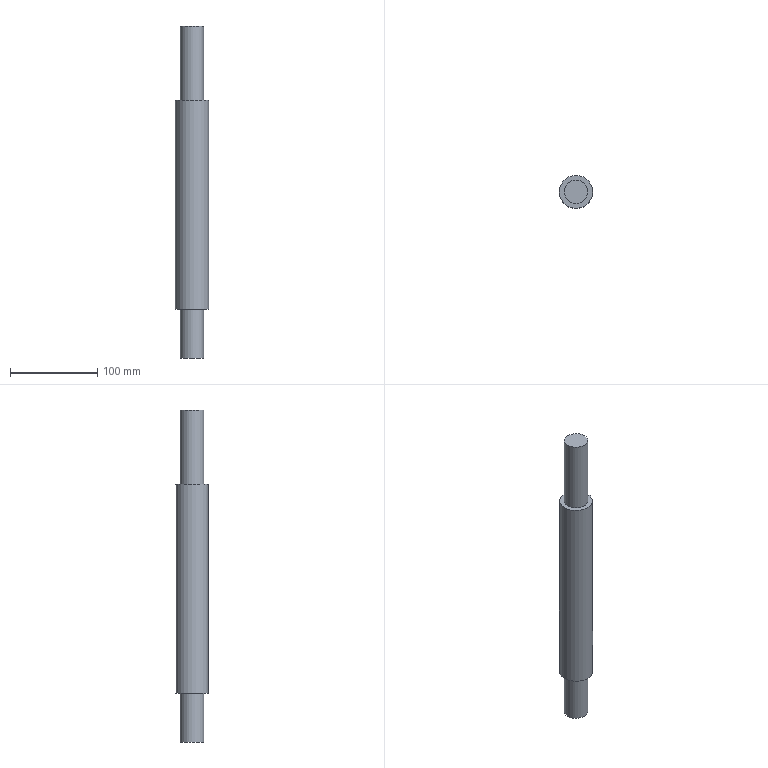Component | NX | SUPPORT_POST | 1 solid | 7 faces | box 38 x 38 x 381 mm | volume 352918 mm3 | plane 4 | cylinder 3 | commonest cylinder face diameters 27 x2 38 x1
STEP:
#1=CARTESIAN_POINT('',(0.,0.,0.));
#2=DIRECTION('',(0.,0.,1.));
#3=DIRECTION('',(1.,0.,0.));
#4=AXIS2_PLACEMENT_3D('',#1,#2,#3);
#5=CARTESIAN_POINT('',(144.,-0.,20.7));
#6=VERTEX_POINT('',#5);
#7=CARTESIAN_POINT('',(125.,-0.,20.7));
#8=DIRECTION('',(0.,0.,1.));
#9=DIRECTION('',(1.,0.,0.));
#10=AXIS2_PLACEMENT_3D('',#7,#8,#9);
#11=CIRCLE('',#10,19.);
#12=CARTESIAN_POINT('',(125.,-0.,20.7));
#13=DIRECTION('',(0.,0.,-1.));
#14=DIRECTION('',(-1.,0.,0.));
#15=AXIS2_PLACEMENT_3D('',#12,#13,#14);
#16=CYLINDRICAL_SURFACE('',#15,19.);
#17=CARTESIAN_POINT('',(9.425,0.));
#18=DIRECTION('',(-1.,0.));
#19=VECTOR('',#18,1.);
#20=LINE('',#17,#19);
#21=(GEOMETRIC_REPRESENTATION_CONTEXT(2)PARAMETRIC_REPRESENTATION_CONTEXT()REPRESENTATION_CONTEXT('',''));
#22=DEFINITIONAL_REPRESENTATION('',(#20),#21);
#23=PCURVE('',#16,#22);
#24=CARTESIAN_POINT('',(125.,-0.,20.7));
#25=DIRECTION('',(0.,0.,1.));
#26=DIRECTION('',(1.,0.,0.));
#27=AXIS2_PLACEMENT_3D('',#24,#25,#26);
#28=PLANE('',#27);
#29=CARTESIAN_POINT('',(0.,0.));
#30=DIRECTION('',(1.,0.));
#31=AXIS2_PLACEMENT_2D('',#29,#30);
#32=CIRCLE('',#31,19.);
#33=(GEOMETRIC_REPRESENTATION_CONTEXT(2)PARAMETRIC_REPRESENTATION_CONTEXT()REPRESENTATION_CONTEXT('',''));
#34=DEFINITIONAL_REPRESENTATION('',(#32),#33);
#35=PCURVE('',#28,#34);
#36=SURFACE_CURVE('',#11,(#23,#35),.PCURVE_S1.);
#37=EDGE_CURVE('',#6,#6,#36,.T.);
#38=ORIENTED_EDGE('',*,*,#37,.F.);
#39=CARTESIAN_POINT('',(144.,-0.,-219.3));
#40=VERTEX_POINT('',#39);
#41=CARTESIAN_POINT('',(144.,-0.,20.7));
#42=CARTESIAN_POINT('',(144.,-0.,-219.3));
#43=B_SPLINE_CURVE_WITH_KNOTS('',1,(#41,#42),.UNSPECIFIED.,.F.,.F.,(2,2),(0.,240.),.PIECEWISE_BEZIER_KNOTS.);
#44=CARTESIAN_POINT('',(9.425,0.));
#45=DIRECTION('',(0.,1.));
#46=VECTOR('',#45,1.);
#47=LINE('',#44,#46);
#48=(GEOMETRIC_REPRESENTATION_CONTEXT(2)PARAMETRIC_REPRESENTATION_CONTEXT()REPRESENTATION_CONTEXT('',''));
#49=DEFINITIONAL_REPRESENTATION('',(#47),#48);
#50=PCURVE('',#16,#49);
#51=CARTESIAN_POINT('',(3.142,0.));
#52=DIRECTION('',(0.,1.));
#53=VECTOR('',#52,1.);
#54=LINE('',#51,#53);
#55=(GEOMETRIC_REPRESENTATION_CONTEXT(2)PARAMETRIC_REPRESENTATION_CONTEXT()REPRESENTATION_CONTEXT('',''));
#56=DEFINITIONAL_REPRESENTATION('',(#54),#55);
#57=PCURVE('',#16,#56);
#58=SEAM_CURVE('',#43,(#50,#57),.PCURVE_S1.);
#59=EDGE_CURVE('',#6,#40,#58,.T.);
#60=ORIENTED_EDGE('',*,*,#59,.T.);
#61=CARTESIAN_POINT('',(125.,-0.,-219.3));
#62=DIRECTION('',(0.,0.,1.));
#63=DIRECTION('',(1.,0.,0.));
#64=AXIS2_PLACEMENT_3D('',#61,#62,#63);
#65=CIRCLE('',#64,19.);
#66=CARTESIAN_POINT('',(9.425,240.));
#67=DIRECTION('',(-1.,0.));
#68=VECTOR('',#67,1.);
#69=LINE('',#66,#68);
#70=(GEOMETRIC_REPRESENTATION_CONTEXT(2)PARAMETRIC_REPRESENTATION_CONTEXT()REPRESENTATION_CONTEXT('',''));
#71=DEFINITIONAL_REPRESENTATION('',(#69),#70);
#72=PCURVE('',#16,#71);
#73=CARTESIAN_POINT('',(125.,-0.,-219.3));
#74=DIRECTION('',(0.,0.,1.));
#75=DIRECTION('',(1.,0.,0.));
#76=AXIS2_PLACEMENT_3D('',#73,#74,#75);
#77=PLANE('',#76);
#78=CARTESIAN_POINT('',(0.,0.));
#79=DIRECTION('',(1.,0.));
#80=AXIS2_PLACEMENT_2D('',#78,#79);
#81=CIRCLE('',#80,19.);
#82=(GEOMETRIC_REPRESENTATION_CONTEXT(2)PARAMETRIC_REPRESENTATION_CONTEXT()REPRESENTATION_CONTEXT('',''));
#83=DEFINITIONAL_REPRESENTATION('',(#81),#82);
#84=PCURVE('',#77,#83);
#85=SURFACE_CURVE('',#65,(#72,#84),.PCURVE_S1.);
#86=EDGE_CURVE('',#40,#40,#85,.T.);
#87=ORIENTED_EDGE('',*,*,#86,.T.);
#88=ORIENTED_EDGE('',*,*,#59,.F.);
#89=EDGE_LOOP('',(#38,#60,#87,#88));
#90=FACE_BOUND('',#89,.T.);
#91=ADVANCED_FACE('',(#90),#16,.T.);
#92=CARTESIAN_POINT('',(138.5,-0.,20.7));
#93=VERTEX_POINT('',#92);
#94=CARTESIAN_POINT('',(125.,-0.,20.7));
#95=DIRECTION('',(0.,0.,1.));
#96=DIRECTION('',(1.,0.,0.));
#97=AXIS2_PLACEMENT_3D('',#94,#95,#96);
#98=CIRCLE('',#97,13.5);
#99=CARTESIAN_POINT('',(0.,0.));
#100=DIRECTION('',(1.,0.));
#101=AXIS2_PLACEMENT_2D('',#99,#100);
#102=CIRCLE('',#101,13.5);
#103=(GEOMETRIC_REPRESENTATION_CONTEXT(2)PARAMETRIC_REPRESENTATION_CONTEXT()REPRESENTATION_CONTEXT('',''));
#104=DEFINITIONAL_REPRESENTATION('',(#102),#103);
#105=PCURVE('',#28,#104);
#106=CARTESIAN_POINT('',(125.,-0.,105.7));
#107=DIRECTION('',(0.,0.,-1.));
#108=DIRECTION('',(-1.,0.,0.));
#109=AXIS2_PLACEMENT_3D('',#106,#107,#108);
#110=CYLINDRICAL_SURFACE('',#109,13.5);
#111=CARTESIAN_POINT('',(9.425,85.));
#112=DIRECTION('',(-1.,0.));
#113=VECTOR('',#112,1.);
#114=LINE('',#111,#113);
#115=(GEOMETRIC_REPRESENTATION_CONTEXT(2)PARAMETRIC_REPRESENTATION_CONTEXT()REPRESENTATION_CONTEXT('',''));
#116=DEFINITIONAL_REPRESENTATION('',(#114),#115);
#117=PCURVE('',#110,#116);
#118=SURFACE_CURVE('',#98,(#105,#117),.PCURVE_S1.);
#119=EDGE_CURVE('',#93,#93,#118,.T.);
#120=ORIENTED_EDGE('',*,*,#119,.F.);
#121=EDGE_LOOP('',(#120));
#122=FACE_BOUND('',#121,.T.);
#123=ORIENTED_EDGE('',*,*,#37,.T.);
#124=EDGE_LOOP('',(#123));
#125=FACE_BOUND('',#124,.T.);
#126=ADVANCED_FACE('',(#122,#125),#28,.T.);
#127=CARTESIAN_POINT('',(138.5,-0.,-219.3));
#128=VERTEX_POINT('',#127);
#129=CARTESIAN_POINT('',(125.,-0.,-219.3));
#130=DIRECTION('',(0.,0.,-1.));
#131=DIRECTION('',(1.,0.,0.));
#132=AXIS2_PLACEMENT_3D('',#129,#130,#131);
#133=CIRCLE('',#132,13.5);
#134=CARTESIAN_POINT('',(13.5,0.));
#135=CARTESIAN_POINT('',(13.5,-23.383));
#136=CARTESIAN_POINT('',(-6.75,-11.691));
#137=CARTESIAN_POINT('',(-27.,-0.));
#138=CARTESIAN_POINT('',(-6.75,11.691));
#139=CARTESIAN_POINT('',(13.5,23.383));
#140=CARTESIAN_POINT('',(13.5,0.));
#141=(BOUNDED_CURVE()B_SPLINE_CURVE(2,(#134,#135,#136,#137,#138,#139,#140),.UNSPECIFIED.,.T.,.F.)B_SPLINE_CURVE_WITH_KNOTS((1,2,2,2,2,1),(-2.094,0.,2.094,4.189,6.283,8.378),.UNSPECIFIED.)CURVE()GEOMETRIC_REPRESENTATION_ITEM()RATIONAL_B_SPLINE_CURVE((1.,0.5,1.,0.5,1.,0.5,1.))REPRESENTATION_ITEM(''));
#142=(GEOMETRIC_REPRESENTATION_CONTEXT(2)PARAMETRIC_REPRESENTATION_CONTEXT()REPRESENTATION_CONTEXT('',''));
#143=DEFINITIONAL_REPRESENTATION('',(#141),#142);
#144=PCURVE('',#77,#143);
#145=CARTESIAN_POINT('',(125.,-0.,-275.3));
#146=DIRECTION('',(0.,0.,1.));
#147=DIRECTION('',(1.,0.,0.));
#148=AXIS2_PLACEMENT_3D('',#145,#146,#147);
#149=CYLINDRICAL_SURFACE('',#148,13.5);
#150=CARTESIAN_POINT('',(6.283,56.));
#151=DIRECTION('',(-1.,0.));
#152=VECTOR('',#151,1.);
#153=LINE('',#150,#152);
#154=(GEOMETRIC_REPRESENTATION_CONTEXT(2)PARAMETRIC_REPRESENTATION_CONTEXT()REPRESENTATION_CONTEXT('',''));
#155=DEFINITIONAL_REPRESENTATION('',(#153),#154);
#156=PCURVE('',#149,#155);
#157=SURFACE_CURVE('',#133,(#144,#156),.PCURVE_S1.);
#158=EDGE_CURVE('',#128,#128,#157,.T.);
#159=ORIENTED_EDGE('',*,*,#158,.F.);
#160=EDGE_LOOP('',(#159));
#161=FACE_BOUND('',#160,.T.);
#162=ORIENTED_EDGE('',*,*,#86,.F.);
#163=EDGE_LOOP('',(#162));
#164=FACE_BOUND('',#163,.T.);
#165=ADVANCED_FACE('',(#161,#164),#77,.F.);
#166=CARTESIAN_POINT('',(138.5,-0.,105.7));
#167=VERTEX_POINT('',#166);
#168=CARTESIAN_POINT('',(125.,-0.,105.7));
#169=DIRECTION('',(0.,0.,1.));
#170=DIRECTION('',(1.,0.,0.));
#171=AXIS2_PLACEMENT_3D('',#168,#169,#170);
#172=CIRCLE('',#171,13.5);
#173=CARTESIAN_POINT('',(9.425,0.));
#174=DIRECTION('',(-1.,0.));
#175=VECTOR('',#174,1.);
#176=LINE('',#173,#175);
#177=(GEOMETRIC_REPRESENTATION_CONTEXT(2)PARAMETRIC_REPRESENTATION_CONTEXT()REPRESENTATION_CONTEXT('',''));
#178=DEFINITIONAL_REPRESENTATION('',(#176),#177);
#179=PCURVE('',#110,#178);
#180=CARTESIAN_POINT('',(125.,-0.,105.7));
#181=DIRECTION('',(0.,0.,1.));
#182=DIRECTION('',(1.,0.,0.));
#183=AXIS2_PLACEMENT_3D('',#180,#181,#182);
#184=PLANE('',#183);
#185=CARTESIAN_POINT('',(0.,0.));
#186=DIRECTION('',(1.,0.));
#187=AXIS2_PLACEMENT_2D('',#185,#186);
#188=CIRCLE('',#187,13.5);
#189=(GEOMETRIC_REPRESENTATION_CONTEXT(2)PARAMETRIC_REPRESENTATION_CONTEXT()REPRESENTATION_CONTEXT('',''));
#190=DEFINITIONAL_REPRESENTATION('',(#188),#189);
#191=PCURVE('',#184,#190);
#192=SURFACE_CURVE('',#172,(#179,#191),.PCURVE_S1.);
#193=EDGE_CURVE('',#167,#167,#192,.T.);
#194=ORIENTED_EDGE('',*,*,#193,.F.);
#195=CARTESIAN_POINT('',(138.5,-0.,105.7));
#196=CARTESIAN_POINT('',(138.5,-0.,20.7));
#197=B_SPLINE_CURVE_WITH_KNOTS('',1,(#195,#196),.UNSPECIFIED.,.F.,.F.,(2,2),(0.,85.),.PIECEWISE_BEZIER_KNOTS.);
#198=CARTESIAN_POINT('',(9.425,0.));
#199=DIRECTION('',(0.,1.));
#200=VECTOR('',#199,1.);
#201=LINE('',#198,#200);
#202=(GEOMETRIC_REPRESENTATION_CONTEXT(2)PARAMETRIC_REPRESENTATION_CONTEXT()REPRESENTATION_CONTEXT('',''));
#203=DEFINITIONAL_REPRESENTATION('',(#201),#202);
#204=PCURVE('',#110,#203);
#205=CARTESIAN_POINT('',(3.142,0.));
#206=DIRECTION('',(0.,1.));
#207=VECTOR('',#206,1.);
#208=LINE('',#205,#207);
#209=(GEOMETRIC_REPRESENTATION_CONTEXT(2)PARAMETRIC_REPRESENTATION_CONTEXT()REPRESENTATION_CONTEXT('',''));
#210=DEFINITIONAL_REPRESENTATION('',(#208),#209);
#211=PCURVE('',#110,#210);
#212=SEAM_CURVE('',#197,(#204,#211),.PCURVE_S1.);
#213=EDGE_CURVE('',#167,#93,#212,.T.);
#214=ORIENTED_EDGE('',*,*,#213,.T.);
#215=ORIENTED_EDGE('',*,*,#119,.T.);
#216=ORIENTED_EDGE('',*,*,#213,.F.);
#217=EDGE_LOOP('',(#194,#214,#215,#216));
#218=FACE_BOUND('',#217,.T.);
#219=ADVANCED_FACE('',(#218),#110,.T.);
#220=ORIENTED_EDGE('',*,*,#193,.T.);
#221=EDGE_LOOP('',(#220));
#222=FACE_BOUND('',#221,.T.);
#223=ADVANCED_FACE('',(#222),#184,.T.);
#224=CARTESIAN_POINT('',(138.5,-0.,-275.3));
#225=VERTEX_POINT('',#224);
#226=CARTESIAN_POINT('',(125.,-0.,-275.3));
#227=DIRECTION('',(0.,0.,-1.));
#228=DIRECTION('',(1.,0.,0.));
#229=AXIS2_PLACEMENT_3D('',#226,#227,#228);
#230=CIRCLE('',#229,13.5);
#231=CARTESIAN_POINT('',(6.283,0.));
#232=DIRECTION('',(-1.,0.));
#233=VECTOR('',#232,1.);
#234=LINE('',#231,#233);
#235=(GEOMETRIC_REPRESENTATION_CONTEXT(2)PARAMETRIC_REPRESENTATION_CONTEXT()REPRESENTATION_CONTEXT('',''));
#236=DEFINITIONAL_REPRESENTATION('',(#234),#235);
#237=PCURVE('',#149,#236);
#238=CARTESIAN_POINT('',(125.,-0.,-275.3));
#239=DIRECTION('',(0.,0.,-1.));
#240=DIRECTION('',(-1.,0.,0.));
#241=AXIS2_PLACEMENT_3D('',#238,#239,#240);
#242=PLANE('',#241);
#243=CARTESIAN_POINT('',(0.,0.));
#244=DIRECTION('',(-1.,0.));
#245=AXIS2_PLACEMENT_2D('',#243,#244);
#246=CIRCLE('',#245,13.5);
#247=(GEOMETRIC_REPRESENTATION_CONTEXT(2)PARAMETRIC_REPRESENTATION_CONTEXT()REPRESENTATION_CONTEXT('',''));
#248=DEFINITIONAL_REPRESENTATION('',(#246),#247);
#249=PCURVE('',#242,#248);
#250=SURFACE_CURVE('',#230,(#237,#249),.PCURVE_S1.);
#251=EDGE_CURVE('',#225,#225,#250,.T.);
#252=ORIENTED_EDGE('',*,*,#251,.F.);
#253=CARTESIAN_POINT('',(138.5,-0.,-275.3));
#254=CARTESIAN_POINT('',(138.5,-0.,-219.3));
#255=B_SPLINE_CURVE_WITH_KNOTS('',1,(#253,#254),.UNSPECIFIED.,.F.,.F.,(2,2),(0.,56.),.PIECEWISE_BEZIER_KNOTS.);
#256=CARTESIAN_POINT('',(6.283,0.));
#257=DIRECTION('',(0.,1.));
#258=VECTOR('',#257,1.);
#259=LINE('',#256,#258);
#260=(GEOMETRIC_REPRESENTATION_CONTEXT(2)PARAMETRIC_REPRESENTATION_CONTEXT()REPRESENTATION_CONTEXT('',''));
#261=DEFINITIONAL_REPRESENTATION('',(#259),#260);
#262=PCURVE('',#149,#261);
#263=CARTESIAN_POINT('',(0.,0.));
#264=DIRECTION('',(0.,1.));
#265=VECTOR('',#264,1.);
#266=LINE('',#263,#265);
#267=(GEOMETRIC_REPRESENTATION_CONTEXT(2)PARAMETRIC_REPRESENTATION_CONTEXT()REPRESENTATION_CONTEXT('',''));
#268=DEFINITIONAL_REPRESENTATION('',(#266),#267);
#269=PCURVE('',#149,#268);
#270=SEAM_CURVE('',#255,(#262,#269),.PCURVE_S1.);
#271=EDGE_CURVE('',#225,#128,#270,.T.);
#272=ORIENTED_EDGE('',*,*,#271,.T.);
#273=ORIENTED_EDGE('',*,*,#158,.T.);
#274=ORIENTED_EDGE('',*,*,#271,.F.);
#275=EDGE_LOOP('',(#252,#272,#273,#274));
#276=FACE_BOUND('',#275,.T.);
#277=ADVANCED_FACE('',(#276),#149,.T.);
#278=ORIENTED_EDGE('',*,*,#251,.T.);
#279=EDGE_LOOP('',(#278));
#280=FACE_BOUND('',#279,.T.);
#281=ADVANCED_FACE('',(#280),#242,.T.);
#282=CLOSED_SHELL('',(#91,#126,#165,#219,#223,#277,#281));
#283=MANIFOLD_SOLID_BREP('',#282);
#284=(LENGTH_UNIT()NAMED_UNIT(*)SI_UNIT(.MILLI.,.METRE.));
#285=UNCERTAINTY_MEASURE_WITH_UNIT(LENGTH_MEASURE(0.00001),#284,'','');
#286=(NAMED_UNIT(*)PLANE_ANGLE_UNIT()SI_UNIT($,.RADIAN.));
#287=(NAMED_UNIT(*)SI_UNIT($,.STERADIAN.)SOLID_ANGLE_UNIT());
#288=(GEOMETRIC_REPRESENTATION_CONTEXT(3)GLOBAL_UNCERTAINTY_ASSIGNED_CONTEXT((#285))GLOBAL_UNIT_ASSIGNED_CONTEXT((#284,#286,#287))REPRESENTATION_CONTEXT('',''));
#289=ADVANCED_BREP_SHAPE_REPRESENTATION('',(#4,#283),#288);